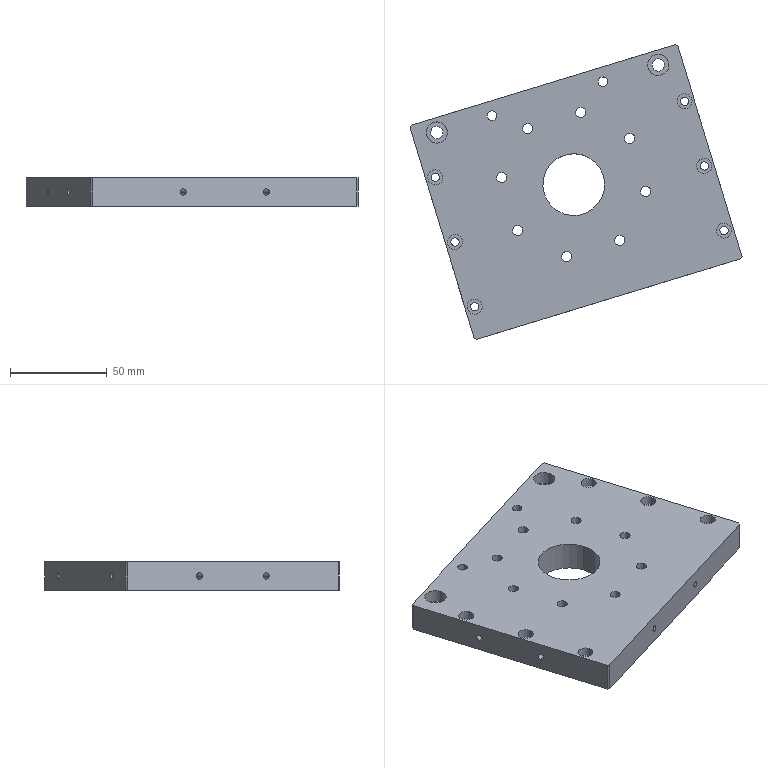Component | SolidWorks | V1ZHXTRotatingPlatformAdapterPlateSB1-1 | 1 solid | 128 faces | box 171.96 x 152.68 x 15 mm | volume 229499 mm3 | cylinder 86 | plane 26 | cone 16 | commonest cylinder face diameters 3.3 x16 10 x16 5.3 x16 7.8 x12 4.3 x12 11 x4 6.4 x4 5 x4 | material 6061 Alloy
build123d program:
from build123d import *

# Parameters (mm, degrees)
SKETCH1_W                                          = 145
SKETCH1_H                                          = 154
BOSS_EXTRUDE1_DEPTH                                = 15
HOLE_SIZE_FOR_HEX_SOCKET_HEAD_CAP_SCRE_D           = 5.3
HOLE_SIZE_FOR_HEX_SOCKET_HEAD_CAP_SCRE_CBORE_D     = 10
HOLE_SIZE_FOR_HEX_SOCKET_HEAD_CAP_SCRE_CBORE_DEPTH = 5.7
SKETCH4_R                                          = 16
CUT_EXTRUDE1_DEPTH                                 = 107.819
CIRPATTERN1_COUNT                                  = 8
SKETCH5_W                                          = 145
SKETCH5_H                                          = 23
CUT_EXTRUDE2_DEPTH                                 = 107.819
SKETCH6_W                                          = 145
SKETCH6_H                                          = 15
CUT_EXTRUDE3_DEPTH                                 = 107.819
SKETCH7_R                                          = 2.5
CUT_EXTRUDE4_DEPTH                                 = 97.567
HOLE_SIZE_ACCORDING_TO_TYPE_2_FOR_HEX_D            = 6.4
HOLE_SIZE_ACCORDING_TO_TYPE_2_FOR_HEX_DEPTH        = 18
HOLE_SIZE_ACCORDING_TO_TYPE_2_FOR_HEX_CBORE_D      = 11
HOLE_SIZE_ACCORDING_TO_TYPE_2_FOR_HEX_CBORE_DEPTH  = 6.8
HOLE_SIZE_ACCORDING_TO_TYPE_2_FOR_HEX_TIP          = 1.923
HOLE_SIZE_BASED_ON_TYPE_3_HEXAGON_2_COUNT          = 2
HOLE_SIZE_BASED_ON_TYPE_3_HEXAGON_2_PITCH          = 35
HOLE_SIZE_BASED_ON_TYPE_3_HEXAGON_3_COUNT          = 2
HOLE_SIZE_BASED_ON_TYPE_3_HEXAGON_3_PITCH          = 70
M4_TAPPED_HOLE1_D                                  = 3.3
M4_TAPPED_HOLE1_DEPTH                              = 12.1
M4_TAPPED_HOLE1_TIP                                = 0.9914
M4_TAPPED_HOLE2_D                                  = 3.3
M4_TAPPED_HOLE2_DEPTH                              = 12.1
M4_TAPPED_HOLE2_TIP                                = 0.9914
M4_TAPPED_HOLE3_D                                  = 3.3
M4_TAPPED_HOLE3_DEPTH                              = 12.1
M4_TAPPED_HOLE3_TIP                                = 0.9914
M4_TAPPED_HOLE4_D                                  = 3.3
M4_TAPPED_HOLE4_DEPTH                              = 12.1
M4_TAPPED_HOLE4_TIP                                = 0.9914
CHAMFER1_SIZE                                      = 1


with BuildPart() as part:
    # Sketch1 → Boss-Extrude1 (new body)
    with BuildSketch(Plane.XY):
        Rectangle(SKETCH1_W, SKETCH1_H)
    extrude(amount=BOSS_EXTRUDE1_DEPTH)

    # Hole Size _for_ Hex Socket Head Cap Scre (through all)
    with Locations(Plane.XY.offset(15)):
        with Locations((34.645, 14.351)):
            hole_size_for_hex_socket_head_cap_scre = CounterBoreHole(HOLE_SIZE_FOR_HEX_SOCKET_HEAD_CAP_SCRE_D / 2, HOLE_SIZE_FOR_HEX_SOCKET_HEAD_CAP_SCRE_CBORE_D / 2, HOLE_SIZE_FOR_HEX_SOCKET_HEAD_CAP_SCRE_CBORE_DEPTH)

    # Sketch4 → Cut-Extrude1 (cut, through all)
    with BuildSketch(Plane.XY.offset(15)):
        Circle(SKETCH4_R)
    extrude(amount=-CUT_EXTRUDE1_DEPTH, mode=Mode.SUBTRACT)

    # CirPattern1: Hole Size _for_ Hex Socket Head Cap Scre ×8 about axis
    cirpattern1_axis = Axis((0, 0, 0), (0, 0, 1))
    for i in range(1, CIRPATTERN1_COUNT):
        add(hole_size_for_hex_socket_head_cap_scre.rotate(cirpattern1_axis, i * 360 / CIRPATTERN1_COUNT), mode=Mode.SUBTRACT)

    # Sketch5 → Cut-Extrude2 (cut, through all)
    with BuildSketch(Plane(origin=(0, 0, 0), x_dir=(-1, 0, 0), z_dir=(0, 0, -1))):
        with Locations((0, -65.5)):
            Rectangle(SKETCH5_W, SKETCH5_H)
    extrude(amount=-CUT_EXTRUDE2_DEPTH, mode=Mode.SUBTRACT)

    # Sketch6 → Cut-Extrude3 (cut, through all)
    with BuildSketch(Plane.XY.offset(15)):
        with Locations((0, 69.5)):
            Rectangle(SKETCH6_W, SKETCH6_H)
    extrude(amount=-CUT_EXTRUDE3_DEPTH, mode=Mode.SUBTRACT)

    # Sketch7 → Cut-Extrude4 (cut, through all)
    with BuildSketch(Plane(origin=(0, 0, 0), x_dir=(-1, 0, 0), z_dir=(0, 0, -1))):
        with Locations((-30, -46.5)):
            Circle(SKETCH7_R)
        with Locations((30, -46.5)):
            Circle(SKETCH7_R)
    extrude(amount=-CUT_EXTRUDE4_DEPTH, mode=Mode.SUBTRACT)

    # Hole Size _ according to_ Type 2 for Hex
    with Locations(Plane(origin=(0, 0, 0), x_dir=(-1, 0, 0), z_dir=(0, 0, -1))):
        with Locations((-60, -46.5), (60, -46.5)):
            CounterBoreHole(HOLE_SIZE_ACCORDING_TO_TYPE_2_FOR_HEX_D / 2, HOLE_SIZE_ACCORDING_TO_TYPE_2_FOR_HEX_CBORE_D / 2, HOLE_SIZE_ACCORDING_TO_TYPE_2_FOR_HEX_CBORE_DEPTH, depth=HOLE_SIZE_ACCORDING_TO_TYPE_2_FOR_HEX_DEPTH)
            with Locations((0, 0, -(HOLE_SIZE_ACCORDING_TO_TYPE_2_FOR_HEX_DEPTH + HOLE_SIZE_ACCORDING_TO_TYPE_2_FOR_HEX_TIP / 2))):  # 118° drill point
                Cone(0, HOLE_SIZE_ACCORDING_TO_TYPE_2_FOR_HEX_D / 2, HOLE_SIZE_ACCORDING_TO_TYPE_2_FOR_HEX_TIP, mode=Mode.SUBTRACT)

    # Sketch10 → Hole Size _ based on_ Type 3 Hexagon Soc (revolve, cut)
    with BuildSketch(Plane(origin=(67.5, 45.5, 0), x_dir=(0, 1, 0), z_dir=(1, 0, 0))):
        Polygon((0, 0), (0, 19.292), (2.15, 18), (2.15, 4.6), (3.9, 4.6), (3.9, 0), align=None)
    hole_size_based_on_type_3_hexagon_soc = revolve(axis=Axis((67.5, 45.5, -6.35), (0, 0, 1)), mode=Mode.SUBTRACT)

    # Hole Size _ based on_ Type 3 Hexagon 2: Hole Size _ based on_ Type 3 Hexagon Soc ×2
    with Locations(*[(0, -i * HOLE_SIZE_BASED_ON_TYPE_3_HEXAGON_2_PITCH, 0) for i in range(1, HOLE_SIZE_BASED_ON_TYPE_3_HEXAGON_2_COUNT)]):
        add(hole_size_based_on_type_3_hexagon_soc, mode=Mode.SUBTRACT)

    # Hole Size _ based on_ Type 3 Hexagon 3: Hole Size _ based on_ Type 3 Hexagon Soc ×2
    with Locations(*[(0, -i * HOLE_SIZE_BASED_ON_TYPE_3_HEXAGON_3_PITCH, 0) for i in range(1, HOLE_SIZE_BASED_ON_TYPE_3_HEXAGON_3_COUNT)]):
        add(hole_size_based_on_type_3_hexagon_soc, mode=Mode.SUBTRACT)

    # Mirror1: Hole Size _ based on_ Type 3 Hexagon Soc across plane
    add(hole_size_based_on_type_3_hexagon_soc.mirror(Plane(origin=(0, 0, 0), x_dir=(0, 0, 1), z_dir=(1, 0, 0))), mode=Mode.SUBTRACT)

    # Mirror1 copy 1 sketch → Mirror1 copy 1 (revolve, cut)
    with BuildSketch(Plane(origin=(-67.5, 10.5, 0), x_dir=(0, 1, 0), z_dir=(-1, 0, 0))):
        Polygon((0, 0), (0, -19.292), (2.15, -18), (2.15, -4.6), (3.9, -4.6), (3.9, 0), align=None)
    revolve(axis=Axis((-67.5, 10.5, -6.35), (0, 0, -1)), mode=Mode.SUBTRACT)

    # Mirror1 copy 2 sketch → Mirror1 copy 2 (revolve, cut)
    with BuildSketch(Plane(origin=(-67.5, -24.5, 0), x_dir=(0, 1, 0), z_dir=(-1, 0, 0))):
        Polygon((0, 0), (0, -19.292), (2.15, -18), (2.15, -4.6), (3.9, -4.6), (3.9, 0), align=None)
    revolve(axis=Axis((-67.5, -24.5, -6.35), (0, 0, -1)), mode=Mode.SUBTRACT)

    # M4 Tapped Hole1
    with Locations(Plane(origin=(0, -54, 0), x_dir=(-1, 0, 0), z_dir=(0, -1, 0))):
        with Locations((-47.5, -7.5), (47.5, -7.5)):
            Hole(M4_TAPPED_HOLE1_D / 2, depth=M4_TAPPED_HOLE1_DEPTH)
            with Locations((0, 0, -(M4_TAPPED_HOLE1_DEPTH + M4_TAPPED_HOLE1_TIP / 2))):  # 118° drill point
                Cone(0, M4_TAPPED_HOLE1_D / 2, M4_TAPPED_HOLE1_TIP, mode=Mode.SUBTRACT)

    # M4 Tapped Hole2
    with Locations(Plane.ZY.offset(72.5)):
        with Locations((7.5, -14), (7.5, 22)):
            Hole(M4_TAPPED_HOLE2_D / 2, depth=M4_TAPPED_HOLE2_DEPTH)
            with Locations((0, 0, -(M4_TAPPED_HOLE2_DEPTH + M4_TAPPED_HOLE2_TIP / 2))):  # 118° drill point
                Cone(0, M4_TAPPED_HOLE2_D / 2, M4_TAPPED_HOLE2_TIP, mode=Mode.SUBTRACT)

    # M4 Tapped Hole3
    with Locations(Plane(origin=(72.5, 0, 0), x_dir=(0, 0, -1), z_dir=(1, 0, 0))):
        with Locations((-7.5, 22), (-7.5, -14)):
            Hole(M4_TAPPED_HOLE3_D / 2, depth=M4_TAPPED_HOLE3_DEPTH)
            with Locations((0, 0, -(M4_TAPPED_HOLE3_DEPTH + M4_TAPPED_HOLE3_TIP / 2))):  # 118° drill point
                Cone(0, M4_TAPPED_HOLE3_D / 2, M4_TAPPED_HOLE3_TIP, mode=Mode.SUBTRACT)

    # M4 Tapped Hole4
    with Locations(Plane(origin=(0, 62, 0), x_dir=(1, 0, 0), z_dir=(0, 1, 0))):
        with Locations((22.5, -7.5), (-22.5, -7.5)):
            Hole(M4_TAPPED_HOLE4_D / 2, depth=M4_TAPPED_HOLE4_DEPTH)
            with Locations((0, 0, -(M4_TAPPED_HOLE4_DEPTH + M4_TAPPED_HOLE4_TIP / 2))):  # 118° drill point
                Cone(0, M4_TAPPED_HOLE4_D / 2, M4_TAPPED_HOLE4_TIP, mode=Mode.SUBTRACT)

    # Chamfer1
    chamfer1_edges = [part.edges().sort_by_distance(p)[0] for p in [
        (72.5, 62, 7.5),
        (72.5, -54, 7.5),
        (-72.5, -54, 7.5),
        (-72.5, 62, 7.5),
    ]]
    chamfer(chamfer1_edges, length=CHAMFER1_SIZE)


solid = part.part

# Placed as in the assembly
solid = solid.moved(Location((176.521, -204.132, 450.239), (-180, 0, -16.968)))